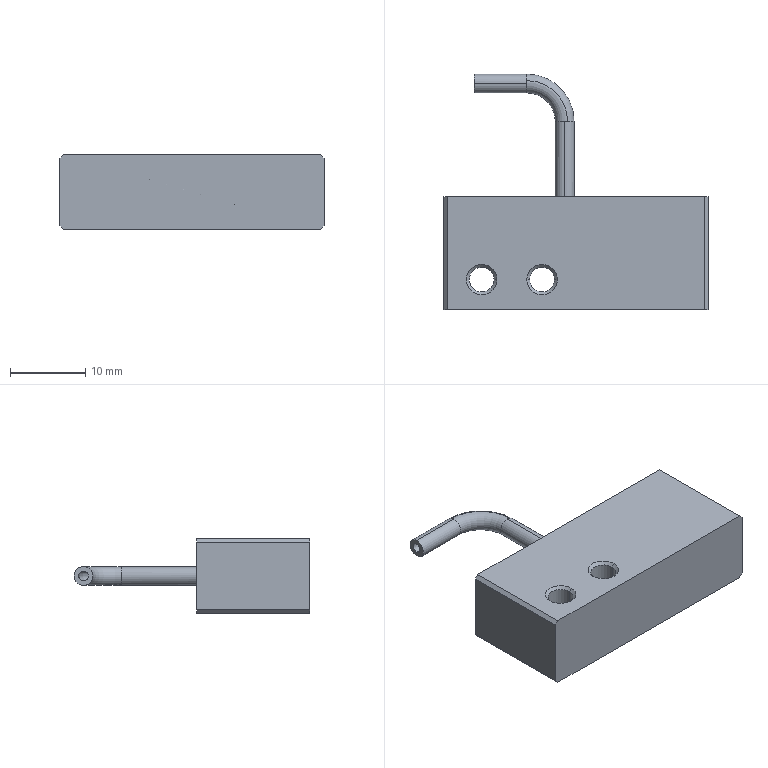CAM job | Mastercam | mm | 13 operations | part box 35 x 31.25 x 10
1. Facing | 23 - 50 平铣刀
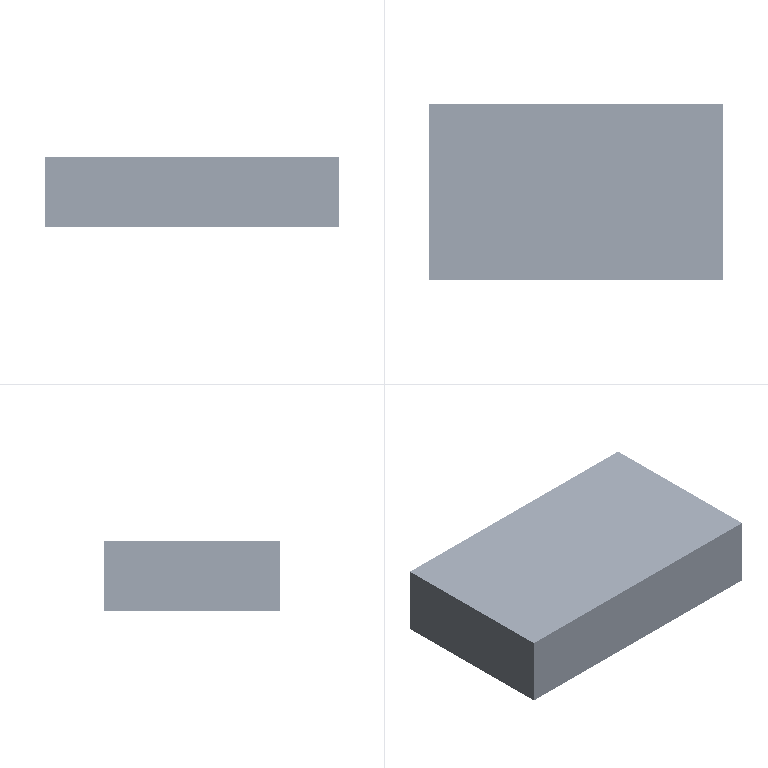2. 2D High Speed (2D Dynamic Mill) | 9 - 10 平铣刀
3. Contour (2D) | 10 - 10 平铣刀
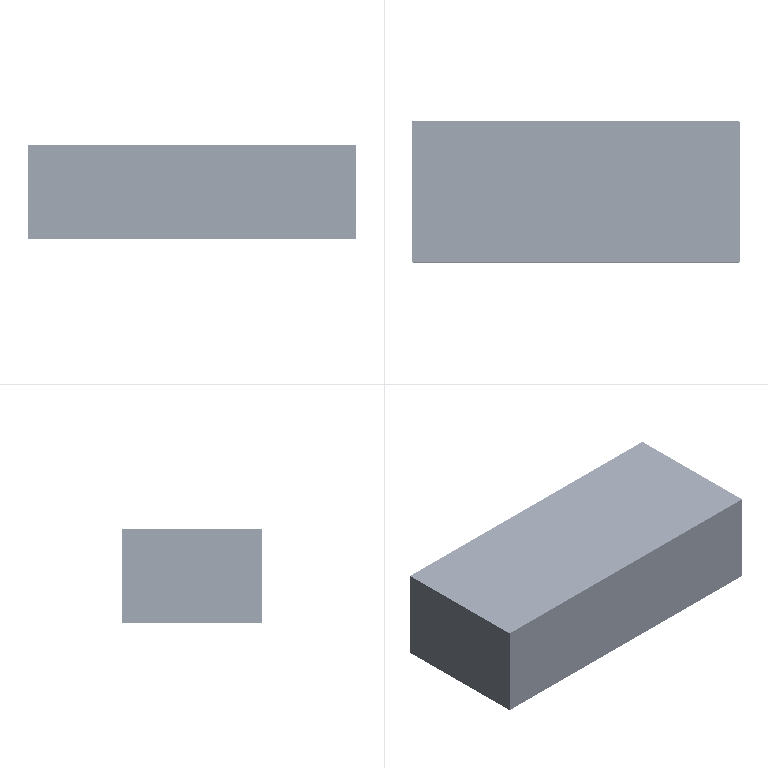4. Facing | 10 - 10 平铣刀
5. Drill/Counterbore | 7 - 6 倒角刀
6. Contour (2D chamfer) | 7 - 6 倒角刀
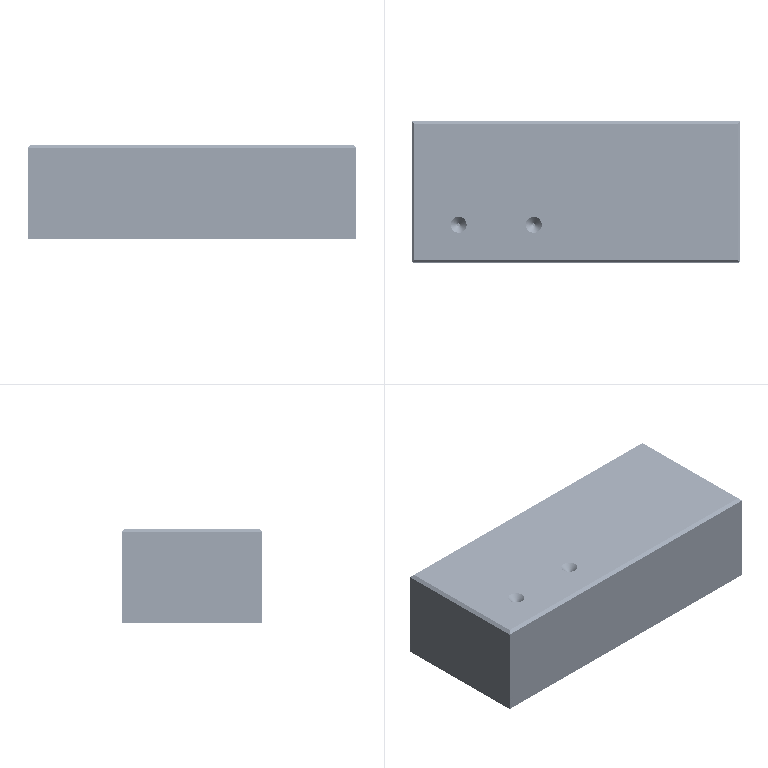7. Contour (2D chamfer) | 7 - 6 倒角刀
8. Facing | 23 - 50 平铣刀
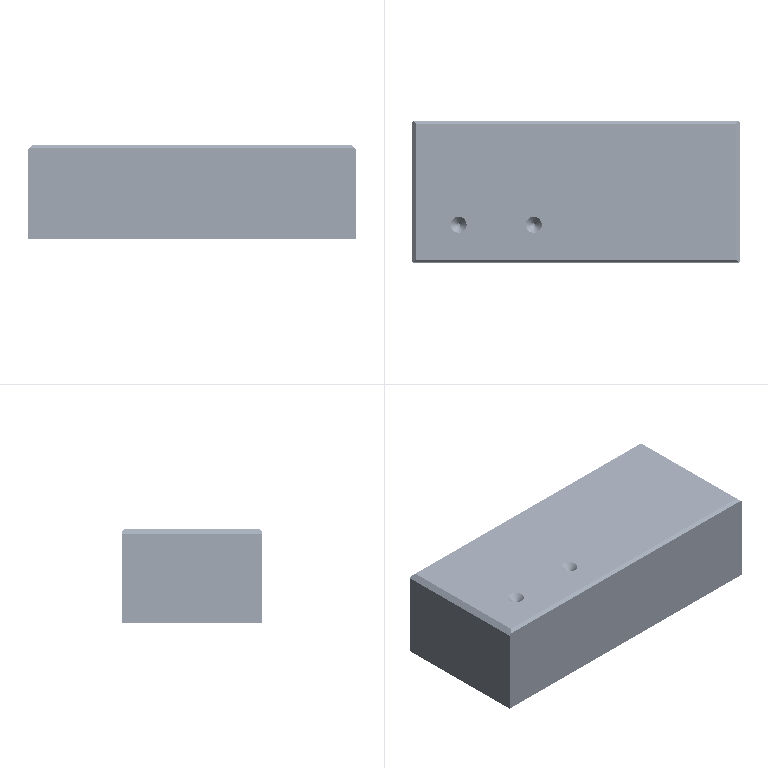9. Facing | 10 - 10 平铣刀
10. Contour (2D chamfer) | 7 - 6 倒角刀
11. Contour (2D chamfer) | 7 - 6 倒角刀
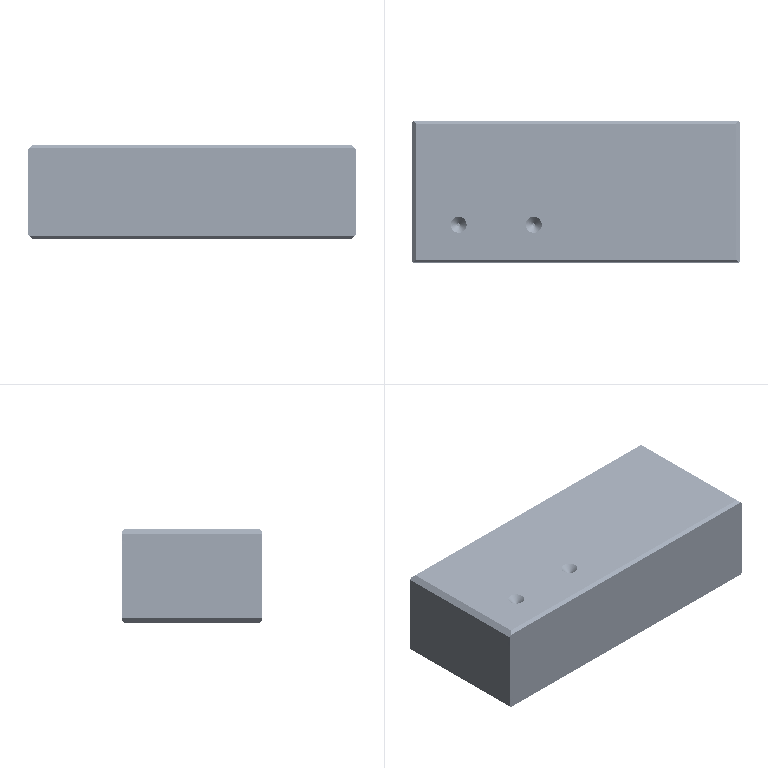12. Drill/Counterbore | 7 - 6 倒角刀
13. Drill/Counterbore | 7 - 6 倒角刀